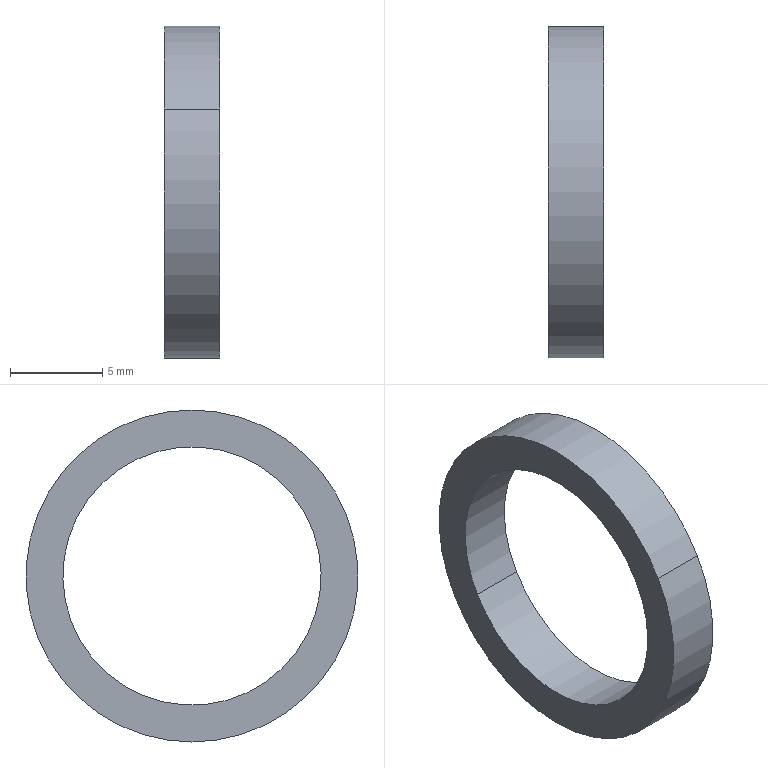Component | SolidWorks | 7mmNut-3 | 1 solid | 6 faces | box 3 x 18 x 18 mm | volume 302 mm3 | cylinder 4 | plane 2 | commonest cylinder face diameters 14 x2 18 x2
build123d program:
from build123d import *

# Parameters (mm, degrees)
SKETCH1_R           = 9
BOSS_EXTRUDE1_DEPTH = 3
CUT_EXTRUDE1_REACH  = 15.077
SKETCH2_R           = 7


with BuildPart() as part:
    # Sketch1 → Boss-Extrude1 (new body)
    with BuildSketch(Plane.XY):
        Circle(SKETCH1_R)
    extrude(amount=BOSS_EXTRUDE1_DEPTH)

    # Sketch2 → Cut-Extrude1 (cut, up to next)
    with BuildSketch(Plane.XY.offset(3), mode=Mode.PRIVATE) as cut_extrude1_sk1:
        Circle(SKETCH2_R)
    cut_extrude1_tool1 = extrude(cut_extrude1_sk1.sketch, amount=-CUT_EXTRUDE1_REACH, mode=Mode.PRIVATE) & part.part
    add(cut_extrude1_tool1.solids().sort_by_distance((0, 0, 3))[0], mode=Mode.SUBTRACT)


solid = part.part

# Placed as in the assembly
solid = solid.moved(Location((125.641, 114.413, 75.777), (0, 90, 0)))